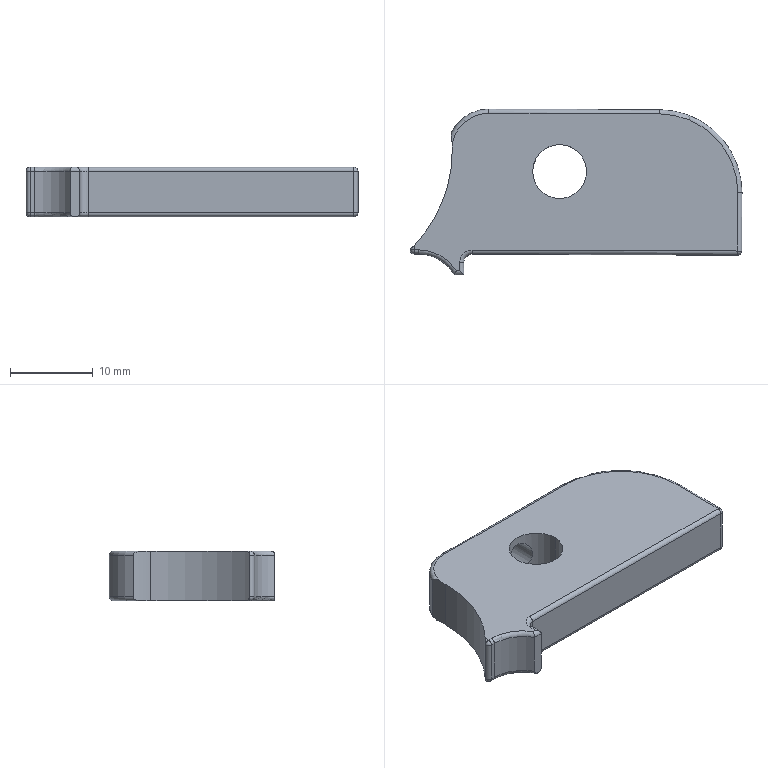Component | SolidWorks | Assembly5.1-1_TailstockAdjustmentSub-Plate.1-2 | 1 solid | 46 faces | volume 3423 mm3 | cylinder 25 | plane 9 | torus 8 | sphere 4 | commonest cylinder face diameters 1 x15 33.112 x2 4 x2 6.5 x2 10 x2 20 x1 2 x1